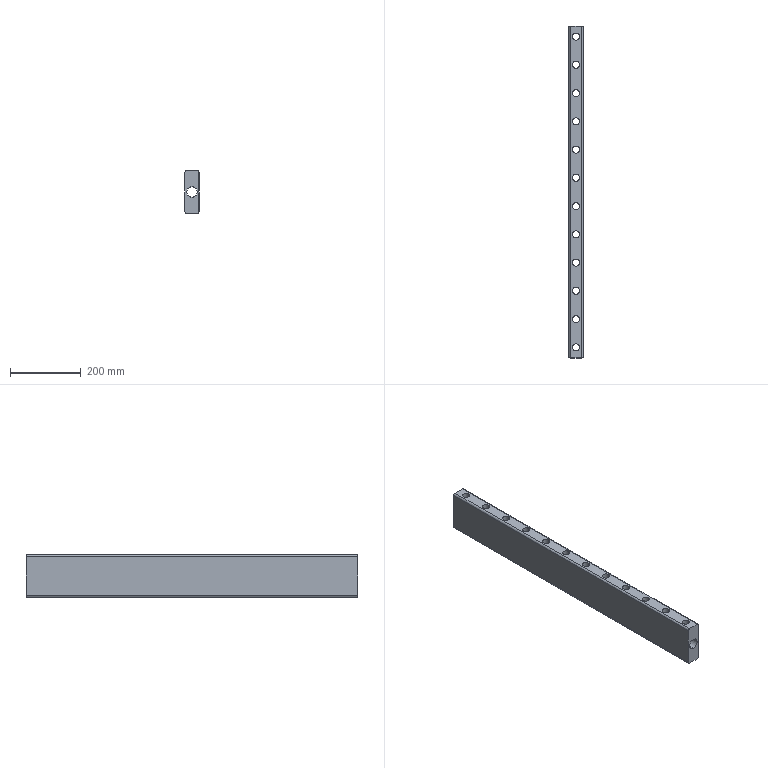Component | SolidWorks | FlipSolderPlate-1 | 1 solid | 62 faces | volume 3481367 mm3 | cylinder 54 | plane 8 | commonest cylinder face diameters 20 x48 10 x4 30 x2 | material Plain Carbon Steel